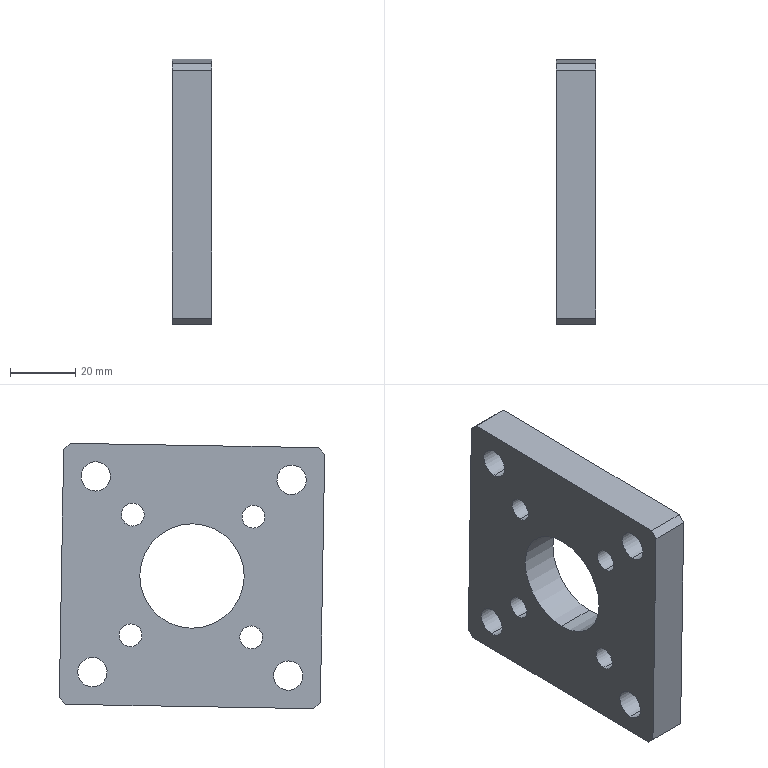Component | SolidWorks | CylinderPlate-1 | 1 solid | 28 faces | box 12 x 81.31 x 81.31 mm | volume 62152 mm3 | cylinder 18 | plane 10 | commonest cylinder face diameters 9 x8 7 x8 32 x2
STEP:
#1=CARTESIAN_POINT('',(37.992,49.965,28.389));
#2=VERTEX_POINT('',#1);
#3=CARTESIAN_POINT('',(37.992,49.971,28.035));
#4=VERTEX_POINT('',#3);
#5=CARTESIAN_POINT('',(37.992,49.968,28.212));
#6=DIRECTION('',(1.,0.,0.));
#7=DIRECTION('',(0.,0.01745,-0.9998));
#8=AXIS2_PLACEMENT_3D('',#5,#6,#7);
#9=CIRCLE('',#8,0.1772);
#10=EDGE_CURVE('',#2,#4,#9,.T.);
#11=ORIENTED_EDGE('',*,*,#10,.T.);
#12=CARTESIAN_POINT('',(37.52,49.971,28.035));
#13=VERTEX_POINT('',#12);
#14=CARTESIAN_POINT('',(37.992,49.971,28.035));
#15=DIRECTION('',(-1.,-0.,-0.));
#16=VECTOR('',#15,39.37);
#17=LINE('',#14,#16);
#18=EDGE_CURVE('',#4,#13,#17,.T.);
#19=ORIENTED_EDGE('',*,*,#18,.T.);
#20=CARTESIAN_POINT('',(37.52,49.965,28.389));
#21=VERTEX_POINT('',#20);
#22=CARTESIAN_POINT('',(37.52,49.968,28.212));
#23=DIRECTION('',(1.,0.,0.));
#24=DIRECTION('',(0.,0.01745,-0.9998));
#25=AXIS2_PLACEMENT_3D('',#22,#23,#24);
#26=CIRCLE('',#25,0.1772);
#27=EDGE_CURVE('',#21,#13,#26,.T.);
#28=ORIENTED_EDGE('',*,*,#27,.F.);
#29=CARTESIAN_POINT('',(37.992,49.965,28.389));
#30=DIRECTION('',(-1.,-0.,-0.));
#31=VECTOR('',#30,39.37);
#32=LINE('',#29,#31);
#33=EDGE_CURVE('',#2,#21,#32,.T.);
#34=ORIENTED_EDGE('',*,*,#33,.F.);
#35=EDGE_LOOP('',(#11,#19,#28,#34));
#36=FACE_OUTER_BOUND('',#35,.T.);
#37=CARTESIAN_POINT('',(37.992,49.968,28.212));
#38=DIRECTION('',(-1.,-0.,-0.));
#39=DIRECTION('',(0.,-0.01745,0.9998));
#40=AXIS2_PLACEMENT_3D('',#37,#38,#39);
#41=CYLINDRICAL_SURFACE('',#40,0.1772);
#42=ADVANCED_FACE('',(#36),#41,.F.);
#43=CARTESIAN_POINT('',(37.992,50.006,26.027));
#44=VERTEX_POINT('',#43);
#45=CARTESIAN_POINT('',(37.992,50.012,25.673));
#46=VERTEX_POINT('',#45);
#47=CARTESIAN_POINT('',(37.992,50.009,25.85));
#48=DIRECTION('',(1.,0.,0.));
#49=DIRECTION('',(0.,0.01745,-0.9998));
#50=AXIS2_PLACEMENT_3D('',#47,#48,#49);
#51=CIRCLE('',#50,0.1772);
#52=EDGE_CURVE('',#44,#46,#51,.T.);
#53=ORIENTED_EDGE('',*,*,#52,.T.);
#54=CARTESIAN_POINT('',(37.52,50.012,25.673));
#55=VERTEX_POINT('',#54);
#56=CARTESIAN_POINT('',(37.992,50.012,25.673));
#57=DIRECTION('',(-1.,-0.,-0.));
#58=VECTOR('',#57,39.37);
#59=LINE('',#56,#58);
#60=EDGE_CURVE('',#46,#55,#59,.T.);
#61=ORIENTED_EDGE('',*,*,#60,.T.);
#62=CARTESIAN_POINT('',(37.52,50.006,26.027));
#63=VERTEX_POINT('',#62);
#64=CARTESIAN_POINT('',(37.52,50.009,25.85));
#65=DIRECTION('',(1.,0.,0.));
#66=DIRECTION('',(0.,0.01745,-0.9998));
#67=AXIS2_PLACEMENT_3D('',#64,#65,#66);
#68=CIRCLE('',#67,0.1772);
#69=EDGE_CURVE('',#63,#55,#68,.T.);
#70=ORIENTED_EDGE('',*,*,#69,.F.);
#71=CARTESIAN_POINT('',(37.992,50.006,26.027));
#72=DIRECTION('',(-1.,-0.,-0.));
#73=VECTOR('',#72,39.37);
#74=LINE('',#71,#73);
#75=EDGE_CURVE('',#44,#63,#74,.T.);
#76=ORIENTED_EDGE('',*,*,#75,.F.);
#77=EDGE_LOOP('',(#53,#61,#70,#76));
#78=FACE_OUTER_BOUND('',#77,.T.);
#79=CARTESIAN_POINT('',(37.992,50.009,25.85));
#80=DIRECTION('',(-1.,-0.,-0.));
#81=DIRECTION('',(0.,-0.01745,0.9998));
#82=AXIS2_PLACEMENT_3D('',#79,#80,#81);
#83=CYLINDRICAL_SURFACE('',#82,0.1772);
#84=ADVANCED_FACE('',(#78),#83,.F.);
#85=CARTESIAN_POINT('',(37.992,52.368,26.069));
#86=VERTEX_POINT('',#85);
#87=CARTESIAN_POINT('',(37.992,52.374,25.714));
#88=VERTEX_POINT('',#87);
#89=CARTESIAN_POINT('',(37.992,52.371,25.891));
#90=DIRECTION('',(1.,0.,0.));
#91=DIRECTION('',(0.,0.01745,-0.9998));
#92=AXIS2_PLACEMENT_3D('',#89,#90,#91);
#93=CIRCLE('',#92,0.1772);
#94=EDGE_CURVE('',#86,#88,#93,.T.);
#95=ORIENTED_EDGE('',*,*,#94,.T.);
#96=CARTESIAN_POINT('',(37.52,52.374,25.714));
#97=VERTEX_POINT('',#96);
#98=CARTESIAN_POINT('',(37.992,52.374,25.714));
#99=DIRECTION('',(-1.,-0.,-0.));
#100=VECTOR('',#99,39.37);
#101=LINE('',#98,#100);
#102=EDGE_CURVE('',#88,#97,#101,.T.);
#103=ORIENTED_EDGE('',*,*,#102,.T.);
#104=CARTESIAN_POINT('',(37.52,52.368,26.069));
#105=VERTEX_POINT('',#104);
#106=CARTESIAN_POINT('',(37.52,52.371,25.891));
#107=DIRECTION('',(1.,0.,0.));
#108=DIRECTION('',(0.,0.01745,-0.9998));
#109=AXIS2_PLACEMENT_3D('',#106,#107,#108);
#110=CIRCLE('',#109,0.1772);
#111=EDGE_CURVE('',#105,#97,#110,.T.);
#112=ORIENTED_EDGE('',*,*,#111,.F.);
#113=CARTESIAN_POINT('',(37.992,52.368,26.069));
#114=DIRECTION('',(-1.,-0.,-0.));
#115=VECTOR('',#114,39.37);
#116=LINE('',#113,#115);
#117=EDGE_CURVE('',#86,#105,#116,.T.);
#118=ORIENTED_EDGE('',*,*,#117,.F.);
#119=EDGE_LOOP('',(#95,#103,#112,#118));
#120=FACE_OUTER_BOUND('',#119,.T.);
#121=CARTESIAN_POINT('',(37.992,52.371,25.891));
#122=DIRECTION('',(-1.,-0.,-0.));
#123=DIRECTION('',(0.,-0.01745,0.9998));
#124=AXIS2_PLACEMENT_3D('',#121,#122,#123);
#125=CYLINDRICAL_SURFACE('',#124,0.1772);
#126=ADVANCED_FACE('',(#120),#125,.F.);
#127=CARTESIAN_POINT('',(37.992,50.426,27.905));
#128=VERTEX_POINT('',#127);
#129=CARTESIAN_POINT('',(37.992,50.431,27.63));
#130=VERTEX_POINT('',#129);
#131=CARTESIAN_POINT('',(37.992,50.429,27.767));
#132=DIRECTION('',(1.,0.,0.));
#133=DIRECTION('',(0.,0.01745,-0.9998));
#134=AXIS2_PLACEMENT_3D('',#131,#132,#133);
#135=CIRCLE('',#134,0.1378);
#136=EDGE_CURVE('',#128,#130,#135,.T.);
#137=ORIENTED_EDGE('',*,*,#136,.T.);
#138=CARTESIAN_POINT('',(37.52,50.431,27.63));
#139=VERTEX_POINT('',#138);
#140=CARTESIAN_POINT('',(37.992,50.431,27.63));
#141=DIRECTION('',(-1.,-0.,-0.));
#142=VECTOR('',#141,39.37);
#143=LINE('',#140,#142);
#144=EDGE_CURVE('',#130,#139,#143,.T.);
#145=ORIENTED_EDGE('',*,*,#144,.T.);
#146=CARTESIAN_POINT('',(37.52,50.426,27.905));
#147=VERTEX_POINT('',#146);
#148=CARTESIAN_POINT('',(37.52,50.429,27.767));
#149=DIRECTION('',(1.,0.,0.));
#150=DIRECTION('',(0.,0.01745,-0.9998));
#151=AXIS2_PLACEMENT_3D('',#148,#149,#150);
#152=CIRCLE('',#151,0.1378);
#153=EDGE_CURVE('',#147,#139,#152,.T.);
#154=ORIENTED_EDGE('',*,*,#153,.F.);
#155=CARTESIAN_POINT('',(37.992,50.426,27.905));
#156=DIRECTION('',(-1.,-0.,-0.));
#157=VECTOR('',#156,39.37);
#158=LINE('',#155,#157);
#159=EDGE_CURVE('',#128,#147,#158,.T.);
#160=ORIENTED_EDGE('',*,*,#159,.F.);
#161=EDGE_LOOP('',(#137,#145,#154,#160));
#162=FACE_OUTER_BOUND('',#161,.T.);
#163=CARTESIAN_POINT('',(37.992,50.429,27.767));
#164=DIRECTION('',(-1.,-0.,-0.));
#165=DIRECTION('',(0.,-0.01745,0.9998));
#166=AXIS2_PLACEMENT_3D('',#163,#164,#165);
#167=CYLINDRICAL_SURFACE('',#166,0.1378);
#168=ADVANCED_FACE('',(#162),#167,.F.);
#169=CARTESIAN_POINT('',(37.992,50.452,26.449));
#170=VERTEX_POINT('',#169);
#171=CARTESIAN_POINT('',(37.992,50.456,26.173));
#172=VERTEX_POINT('',#171);
#173=CARTESIAN_POINT('',(37.992,50.454,26.311));
#174=DIRECTION('',(1.,0.,0.));
#175=DIRECTION('',(0.,0.01745,-0.9998));
#176=AXIS2_PLACEMENT_3D('',#173,#174,#175);
#177=CIRCLE('',#176,0.1378);
#178=EDGE_CURVE('',#170,#172,#177,.T.);
#179=ORIENTED_EDGE('',*,*,#178,.T.);
#180=CARTESIAN_POINT('',(37.52,50.456,26.173));
#181=VERTEX_POINT('',#180);
#182=CARTESIAN_POINT('',(37.992,50.456,26.173));
#183=DIRECTION('',(-1.,-0.,-0.));
#184=VECTOR('',#183,39.37);
#185=LINE('',#182,#184);
#186=EDGE_CURVE('',#172,#181,#185,.T.);
#187=ORIENTED_EDGE('',*,*,#186,.T.);
#188=CARTESIAN_POINT('',(37.52,50.452,26.449));
#189=VERTEX_POINT('',#188);
#190=CARTESIAN_POINT('',(37.52,50.454,26.311));
#191=DIRECTION('',(1.,0.,0.));
#192=DIRECTION('',(0.,0.01745,-0.9998));
#193=AXIS2_PLACEMENT_3D('',#190,#191,#192);
#194=CIRCLE('',#193,0.1378);
#195=EDGE_CURVE('',#189,#181,#194,.T.);
#196=ORIENTED_EDGE('',*,*,#195,.F.);
#197=CARTESIAN_POINT('',(37.992,50.452,26.449));
#198=DIRECTION('',(-1.,-0.,-0.));
#199=VECTOR('',#198,39.37);
#200=LINE('',#197,#199);
#201=EDGE_CURVE('',#170,#189,#200,.T.);
#202=ORIENTED_EDGE('',*,*,#201,.F.);
#203=EDGE_LOOP('',(#179,#187,#196,#202));
#204=FACE_OUTER_BOUND('',#203,.T.);
#205=CARTESIAN_POINT('',(37.992,50.454,26.311));
#206=DIRECTION('',(-1.,-0.,-0.));
#207=DIRECTION('',(0.,-0.01745,0.9998));
#208=AXIS2_PLACEMENT_3D('',#205,#206,#207);
#209=CYLINDRICAL_SURFACE('',#208,0.1378);
#210=ADVANCED_FACE('',(#204),#209,.F.);
#211=CARTESIAN_POINT('',(37.992,51.908,26.474));
#212=VERTEX_POINT('',#211);
#213=CARTESIAN_POINT('',(37.992,51.913,26.199));
#214=VERTEX_POINT('',#213);
#215=CARTESIAN_POINT('',(37.992,51.91,26.336));
#216=DIRECTION('',(1.,0.,0.));
#217=DIRECTION('',(0.,0.01745,-0.9998));
#218=AXIS2_PLACEMENT_3D('',#215,#216,#217);
#219=CIRCLE('',#218,0.1378);
#220=EDGE_CURVE('',#212,#214,#219,.T.);
#221=ORIENTED_EDGE('',*,*,#220,.T.);
#222=CARTESIAN_POINT('',(37.52,51.913,26.199));
#223=VERTEX_POINT('',#222);
#224=CARTESIAN_POINT('',(37.992,51.913,26.199));
#225=DIRECTION('',(-1.,-0.,-0.));
#226=VECTOR('',#225,39.37);
#227=LINE('',#224,#226);
#228=EDGE_CURVE('',#214,#223,#227,.T.);
#229=ORIENTED_EDGE('',*,*,#228,.T.);
#230=CARTESIAN_POINT('',(37.52,51.908,26.474));
#231=VERTEX_POINT('',#230);
#232=CARTESIAN_POINT('',(37.52,51.91,26.336));
#233=DIRECTION('',(1.,0.,0.));
#234=DIRECTION('',(0.,0.01745,-0.9998));
#235=AXIS2_PLACEMENT_3D('',#232,#233,#234);
#236=CIRCLE('',#235,0.1378);
#237=EDGE_CURVE('',#231,#223,#236,.T.);
#238=ORIENTED_EDGE('',*,*,#237,.F.);
#239=CARTESIAN_POINT('',(37.992,51.908,26.474));
#240=DIRECTION('',(-1.,-0.,-0.));
#241=VECTOR('',#240,39.37);
#242=LINE('',#239,#241);
#243=EDGE_CURVE('',#212,#231,#242,.T.);
#244=ORIENTED_EDGE('',*,*,#243,.F.);
#245=EDGE_LOOP('',(#221,#229,#238,#244));
#246=FACE_OUTER_BOUND('',#245,.T.);
#247=CARTESIAN_POINT('',(37.992,51.91,26.336));
#248=DIRECTION('',(-1.,-0.,-0.));
#249=DIRECTION('',(0.,-0.01745,0.9998));
#250=AXIS2_PLACEMENT_3D('',#247,#248,#249);
#251=CYLINDRICAL_SURFACE('',#250,0.1378);
#252=ADVANCED_FACE('',(#246),#251,.F.);
#253=CARTESIAN_POINT('',(37.992,52.327,28.43));
#254=VERTEX_POINT('',#253);
#255=CARTESIAN_POINT('',(37.992,52.333,28.076));
#256=VERTEX_POINT('',#255);
#257=CARTESIAN_POINT('',(37.992,52.33,28.253));
#258=DIRECTION('',(1.,0.,0.));
#259=DIRECTION('',(0.,0.01745,-0.9998));
#260=AXIS2_PLACEMENT_3D('',#257,#258,#259);
#261=CIRCLE('',#260,0.1772);
#262=EDGE_CURVE('',#254,#256,#261,.T.);
#263=ORIENTED_EDGE('',*,*,#262,.T.);
#264=CARTESIAN_POINT('',(37.52,52.333,28.076));
#265=VERTEX_POINT('',#264);
#266=CARTESIAN_POINT('',(37.992,52.333,28.076));
#267=DIRECTION('',(-1.,-0.,-0.));
#268=VECTOR('',#267,39.37);
#269=LINE('',#266,#268);
#270=EDGE_CURVE('',#256,#265,#269,.T.);
#271=ORIENTED_EDGE('',*,*,#270,.T.);
#272=CARTESIAN_POINT('',(37.52,52.327,28.43));
#273=VERTEX_POINT('',#272);
#274=CARTESIAN_POINT('',(37.52,52.33,28.253));
#275=DIRECTION('',(1.,0.,0.));
#276=DIRECTION('',(0.,0.01745,-0.9998));
#277=AXIS2_PLACEMENT_3D('',#274,#275,#276);
#278=CIRCLE('',#277,0.1772);
#279=EDGE_CURVE('',#273,#265,#278,.T.);
#280=ORIENTED_EDGE('',*,*,#279,.F.);
#281=CARTESIAN_POINT('',(37.992,52.327,28.43));
#282=DIRECTION('',(-1.,-0.,-0.));
#283=VECTOR('',#282,39.37);
#284=LINE('',#281,#283);
#285=EDGE_CURVE('',#254,#273,#284,.T.);
#286=ORIENTED_EDGE('',*,*,#285,.F.);
#287=EDGE_LOOP('',(#263,#271,#280,#286));
#288=FACE_OUTER_BOUND('',#287,.T.);
#289=CARTESIAN_POINT('',(37.992,52.33,28.253));
#290=DIRECTION('',(-1.,-0.,-0.));
#291=DIRECTION('',(0.,-0.01745,0.9998));
#292=AXIS2_PLACEMENT_3D('',#289,#290,#291);
#293=CYLINDRICAL_SURFACE('',#292,0.1772);
#294=ADVANCED_FACE('',(#288),#293,.F.);
#295=CARTESIAN_POINT('',(37.992,51.159,27.682));
#296=VERTEX_POINT('',#295);
#297=CARTESIAN_POINT('',(37.992,51.181,26.422));
#298=VERTEX_POINT('',#297);
#299=CARTESIAN_POINT('',(37.992,51.17,27.052));
#300=DIRECTION('',(1.,0.,0.));
#301=DIRECTION('',(0.,0.01745,-0.9998));
#302=AXIS2_PLACEMENT_3D('',#299,#300,#301);
#303=CIRCLE('',#302,0.6299);
#304=EDGE_CURVE('',#296,#298,#303,.T.);
#305=ORIENTED_EDGE('',*,*,#304,.T.);
#306=CARTESIAN_POINT('',(37.52,51.181,26.422));
#307=VERTEX_POINT('',#306);
#308=CARTESIAN_POINT('',(37.992,51.181,26.422));
#309=DIRECTION('',(-1.,-0.,-0.));
#310=VECTOR('',#309,39.37);
#311=LINE('',#308,#310);
#312=EDGE_CURVE('',#298,#307,#311,.T.);
#313=ORIENTED_EDGE('',*,*,#312,.T.);
#314=CARTESIAN_POINT('',(37.52,51.159,27.682));
#315=VERTEX_POINT('',#314);
#316=CARTESIAN_POINT('',(37.52,51.17,27.052));
#317=DIRECTION('',(1.,0.,0.));
#318=DIRECTION('',(0.,0.01745,-0.9998));
#319=AXIS2_PLACEMENT_3D('',#316,#317,#318);
#320=CIRCLE('',#319,0.6299);
#321=EDGE_CURVE('',#315,#307,#320,.T.);
#322=ORIENTED_EDGE('',*,*,#321,.F.);
#323=CARTESIAN_POINT('',(37.992,51.159,27.682));
#324=DIRECTION('',(-1.,-0.,-0.));
#325=VECTOR('',#324,39.37);
#326=LINE('',#323,#325);
#327=EDGE_CURVE('',#296,#315,#326,.T.);
#328=ORIENTED_EDGE('',*,*,#327,.F.);
#329=EDGE_LOOP('',(#305,#313,#322,#328));
#330=FACE_OUTER_BOUND('',#329,.T.);
#331=CARTESIAN_POINT('',(37.992,51.17,27.052));
#332=DIRECTION('',(-1.,-0.,-0.));
#333=DIRECTION('',(0.,-0.01745,0.9998));
#334=AXIS2_PLACEMENT_3D('',#331,#332,#333);
#335=CYLINDRICAL_SURFACE('',#334,0.6299);
#336=ADVANCED_FACE('',(#330),#335,.F.);
#337=CARTESIAN_POINT('',(37.992,51.883,27.931));
#338=VERTEX_POINT('',#337);
#339=CARTESIAN_POINT('',(37.992,51.887,27.655));
#340=VERTEX_POINT('',#339);
#341=CARTESIAN_POINT('',(37.992,51.885,27.793));
#342=DIRECTION('',(1.,0.,0.));
#343=DIRECTION('',(0.,0.01745,-0.9998));
#344=AXIS2_PLACEMENT_3D('',#341,#342,#343);
#345=CIRCLE('',#344,0.1378);
#346=EDGE_CURVE('',#338,#340,#345,.T.);
#347=ORIENTED_EDGE('',*,*,#346,.T.);
#348=CARTESIAN_POINT('',(37.52,51.887,27.655));
#349=VERTEX_POINT('',#348);
#350=CARTESIAN_POINT('',(37.992,51.887,27.655));
#351=DIRECTION('',(-1.,-0.,-0.));
#352=VECTOR('',#351,39.37);
#353=LINE('',#350,#352);
#354=EDGE_CURVE('',#340,#349,#353,.T.);
#355=ORIENTED_EDGE('',*,*,#354,.T.);
#356=CARTESIAN_POINT('',(37.52,51.883,27.931));
#357=VERTEX_POINT('',#356);
#358=CARTESIAN_POINT('',(37.52,51.885,27.793));
#359=DIRECTION('',(1.,0.,0.));
#360=DIRECTION('',(0.,0.01745,-0.9998));
#361=AXIS2_PLACEMENT_3D('',#358,#359,#360);
#362=CIRCLE('',#361,0.1378);
#363=EDGE_CURVE('',#357,#349,#362,.T.);
#364=ORIENTED_EDGE('',*,*,#363,.F.);
#365=CARTESIAN_POINT('',(37.992,51.883,27.931));
#366=DIRECTION('',(-1.,-0.,-0.));
#367=VECTOR('',#366,39.37);
#368=LINE('',#365,#367);
#369=EDGE_CURVE('',#338,#357,#368,.T.);
#370=ORIENTED_EDGE('',*,*,#369,.F.);
#371=EDGE_LOOP('',(#347,#355,#364,#370));
#372=FACE_OUTER_BOUND('',#371,.T.);
#373=CARTESIAN_POINT('',(37.992,51.885,27.793));
#374=DIRECTION('',(-1.,-0.,-0.));
#375=DIRECTION('',(0.,-0.01745,0.9998));
#376=AXIS2_PLACEMENT_3D('',#373,#374,#375);
#377=CYLINDRICAL_SURFACE('',#376,0.1378);
#378=ADVANCED_FACE('',(#372),#377,.F.);
#379=ORIENTED_EDGE('',*,*,#52,.F.);
#380=CARTESIAN_POINT('',(37.992,50.009,25.85));
#381=DIRECTION('',(1.,0.,0.));
#382=DIRECTION('',(0.,0.01745,-0.9998));
#383=AXIS2_PLACEMENT_3D('',#380,#381,#382);
#384=CIRCLE('',#383,0.1772);
#385=EDGE_CURVE('',#46,#44,#384,.T.);
#386=ORIENTED_EDGE('',*,*,#385,.F.);
#387=EDGE_LOOP('',(#379,#386));
#388=FACE_BOUND('',#387,.T.);
#389=ORIENTED_EDGE('',*,*,#136,.F.);
#390=CARTESIAN_POINT('',(37.992,50.429,27.767));
#391=DIRECTION('',(1.,0.,0.));
#392=DIRECTION('',(0.,0.01745,-0.9998));
#393=AXIS2_PLACEMENT_3D('',#390,#391,#392);
#394=CIRCLE('',#393,0.1378);
#395=EDGE_CURVE('',#130,#128,#394,.T.);
#396=ORIENTED_EDGE('',*,*,#395,.F.);
#397=EDGE_LOOP('',(#389,#396));
#398=FACE_BOUND('',#397,.T.);
#399=ORIENTED_EDGE('',*,*,#220,.F.);
#400=CARTESIAN_POINT('',(37.992,51.91,26.336));
#401=DIRECTION('',(1.,0.,0.));
#402=DIRECTION('',(0.,0.01745,-0.9998));
#403=AXIS2_PLACEMENT_3D('',#400,#401,#402);
#404=CIRCLE('',#403,0.1378);
#405=EDGE_CURVE('',#214,#212,#404,.T.);
#406=ORIENTED_EDGE('',*,*,#405,.F.);
#407=EDGE_LOOP('',(#399,#406));
#408=FACE_BOUND('',#407,.T.);
#409=ORIENTED_EDGE('',*,*,#304,.F.);
#410=CARTESIAN_POINT('',(37.992,51.17,27.052));
#411=DIRECTION('',(1.,0.,0.));
#412=DIRECTION('',(0.,0.01745,-0.9998));
#413=AXIS2_PLACEMENT_3D('',#410,#411,#412);
#414=CIRCLE('',#413,0.6299);
#415=EDGE_CURVE('',#298,#296,#414,.T.);
#416=ORIENTED_EDGE('',*,*,#415,.F.);
#417=EDGE_LOOP('',(#409,#416));
#418=FACE_BOUND('',#417,.T.);
#419=CARTESIAN_POINT('',(37.992,52.638,28.652));
#420=VERTEX_POINT('',#419);
#421=CARTESIAN_POINT('',(37.992,49.646,28.6));
#422=VERTEX_POINT('',#421);
#423=CARTESIAN_POINT('',(37.992,52.717,28.654));
#424=DIRECTION('',(0.,-0.9998,-0.01745));
#425=VECTOR('',#424,39.37);
#426=LINE('',#423,#425);
#427=EDGE_CURVE('',#420,#422,#426,.T.);
#428=ORIENTED_EDGE('',*,*,#427,.T.);
#429=CARTESIAN_POINT('',(37.992,49.569,28.52));
#430=VERTEX_POINT('',#429);
#431=CARTESIAN_POINT('',(37.992,49.608,28.56));
#432=DIRECTION('',(0.,-0.6947,-0.7193));
#433=VECTOR('',#432,39.37);
#434=LINE('',#431,#433);
#435=EDGE_CURVE('',#422,#430,#434,.T.);
#436=ORIENTED_EDGE('',*,*,#435,.T.);
#437=CARTESIAN_POINT('',(37.992,49.621,25.528));
#438=VERTEX_POINT('',#437);
#439=CARTESIAN_POINT('',(37.992,49.567,28.599));
#440=DIRECTION('',(-0.,0.01745,-0.9998));
#441=VECTOR('',#440,39.37);
#442=LINE('',#439,#441);
#443=EDGE_CURVE('',#430,#438,#442,.T.);
#444=ORIENTED_EDGE('',*,*,#443,.T.);
#445=CARTESIAN_POINT('',(37.992,49.701,25.451));
#446=VERTEX_POINT('',#445);
#447=CARTESIAN_POINT('',(37.992,49.661,25.49));
#448=DIRECTION('',(-0.,0.7193,-0.6947));
#449=VECTOR('',#448,39.37);
#450=LINE('',#447,#449);
#451=EDGE_CURVE('',#438,#446,#450,.T.);
#452=ORIENTED_EDGE('',*,*,#451,.T.);
#453=CARTESIAN_POINT('',(37.992,52.693,25.503));
#454=VERTEX_POINT('',#453);
#455=CARTESIAN_POINT('',(37.992,52.772,25.505));
#456=DIRECTION('',(-0.,0.9998,0.01745));
#457=VECTOR('',#456,39.37);
#458=LINE('',#455,#457);
#459=EDGE_CURVE('',#446,#454,#458,.T.);
#460=ORIENTED_EDGE('',*,*,#459,.T.);
#461=CARTESIAN_POINT('',(37.992,52.77,25.583));
#462=VERTEX_POINT('',#461);
#463=CARTESIAN_POINT('',(37.992,52.732,25.543));
#464=DIRECTION('',(-0.,0.6947,0.7193));
#465=VECTOR('',#464,39.37);
#466=LINE('',#463,#465);
#467=EDGE_CURVE('',#454,#462,#466,.T.);
#468=ORIENTED_EDGE('',*,*,#467,.T.);
#469=CARTESIAN_POINT('',(37.992,52.718,28.575));
#470=VERTEX_POINT('',#469);
#471=CARTESIAN_POINT('',(37.992,52.717,28.654));
#472=DIRECTION('',(0.,-0.01745,0.9998));
#473=VECTOR('',#472,39.37);
#474=LINE('',#471,#473);
#475=EDGE_CURVE('',#462,#470,#474,.T.);
#476=ORIENTED_EDGE('',*,*,#475,.T.);
#477=CARTESIAN_POINT('',(37.992,52.678,28.614));
#478=DIRECTION('',(0.,-0.7193,0.6947));
#479=VECTOR('',#478,39.37);
#480=LINE('',#477,#479);
#481=EDGE_CURVE('',#470,#420,#480,.T.);
#482=ORIENTED_EDGE('',*,*,#481,.T.);
#483=EDGE_LOOP('',(#428,#436,#444,#452,#460,#468,#476,#482));
#484=FACE_OUTER_BOUND('',#483,.T.);
#485=ORIENTED_EDGE('',*,*,#346,.F.);
#486=CARTESIAN_POINT('',(37.992,51.885,27.793));
#487=DIRECTION('',(1.,0.,0.));
#488=DIRECTION('',(0.,0.01745,-0.9998));
#489=AXIS2_PLACEMENT_3D('',#486,#487,#488);
#490=CIRCLE('',#489,0.1378);
#491=EDGE_CURVE('',#340,#338,#490,.T.);
#492=ORIENTED_EDGE('',*,*,#491,.F.);
#493=EDGE_LOOP('',(#485,#492));
#494=FACE_BOUND('',#493,.T.);
#495=ORIENTED_EDGE('',*,*,#262,.F.);
#496=CARTESIAN_POINT('',(37.992,52.33,28.253));
#497=DIRECTION('',(1.,0.,0.));
#498=DIRECTION('',(0.,0.01745,-0.9998));
#499=AXIS2_PLACEMENT_3D('',#496,#497,#498);
#500=CIRCLE('',#499,0.1772);
#501=EDGE_CURVE('',#256,#254,#500,.T.);
#502=ORIENTED_EDGE('',*,*,#501,.F.);
#503=EDGE_LOOP('',(#495,#502));
#504=FACE_BOUND('',#503,.T.);
#505=ORIENTED_EDGE('',*,*,#178,.F.);
#506=CARTESIAN_POINT('',(37.992,50.454,26.311));
#507=DIRECTION('',(1.,0.,0.));
#508=DIRECTION('',(0.,0.01745,-0.9998));
#509=AXIS2_PLACEMENT_3D('',#506,#507,#508);
#510=CIRCLE('',#509,0.1378);
#511=EDGE_CURVE('',#172,#170,#510,.T.);
#512=ORIENTED_EDGE('',*,*,#511,.F.);
#513=EDGE_LOOP('',(#505,#512));
#514=FACE_BOUND('',#513,.T.);
#515=ORIENTED_EDGE('',*,*,#94,.F.);
#516=CARTESIAN_POINT('',(37.992,52.371,25.891));
#517=DIRECTION('',(1.,0.,0.));
#518=DIRECTION('',(0.,0.01745,-0.9998));
#519=AXIS2_PLACEMENT_3D('',#516,#517,#518);
#520=CIRCLE('',#519,0.1772);
#521=EDGE_CURVE('',#88,#86,#520,.T.);
#522=ORIENTED_EDGE('',*,*,#521,.F.);
#523=EDGE_LOOP('',(#515,#522));
#524=FACE_BOUND('',#523,.T.);
#525=ORIENTED_EDGE('',*,*,#10,.F.);
#526=CARTESIAN_POINT('',(37.992,49.968,28.212));
#527=DIRECTION('',(1.,0.,0.));
#528=DIRECTION('',(0.,0.01745,-0.9998));
#529=AXIS2_PLACEMENT_3D('',#526,#527,#528);
#530=CIRCLE('',#529,0.1772);
#531=EDGE_CURVE('',#4,#2,#530,.T.);
#532=ORIENTED_EDGE('',*,*,#531,.F.);
#533=EDGE_LOOP('',(#525,#532));
#534=FACE_BOUND('',#533,.T.);
#535=CARTESIAN_POINT('',(37.992,51.17,27.052));
#536=DIRECTION('',(1.,0.,0.));
#537=DIRECTION('',(-0.,0.01745,-0.9998));
#538=AXIS2_PLACEMENT_3D('',#535,#536,#537);
#539=PLANE('',#538);
#540=ADVANCED_FACE('',(#388,#398,#408,#418,#484,#494,#504,#514,#524,#534),#539,.T.);
#541=CARTESIAN_POINT('',(37.52,49.569,28.52));
#542=VERTEX_POINT('',#541);
#543=CARTESIAN_POINT('',(37.52,49.621,25.528));
#544=VERTEX_POINT('',#543);
#545=CARTESIAN_POINT('',(37.52,49.567,28.599));
#546=DIRECTION('',(-0.,0.01745,-0.9998));
#547=VECTOR('',#546,39.37);
#548=LINE('',#545,#547);
#549=EDGE_CURVE('',#542,#544,#548,.T.);
#550=ORIENTED_EDGE('',*,*,#549,.F.);
#551=CARTESIAN_POINT('',(37.52,49.646,28.6));
#552=VERTEX_POINT('',#551);
#553=CARTESIAN_POINT('',(37.52,49.569,28.52));
#554=DIRECTION('',(-0.,0.6947,0.7193));
#555=VECTOR('',#554,39.37);
#556=LINE('',#553,#555);
#557=EDGE_CURVE('',#542,#552,#556,.T.);
#558=ORIENTED_EDGE('',*,*,#557,.T.);
#559=CARTESIAN_POINT('',(37.52,52.638,28.652));
#560=VERTEX_POINT('',#559);
#561=CARTESIAN_POINT('',(37.52,52.717,28.654));
#562=DIRECTION('',(0.,-0.9998,-0.01745));
#563=VECTOR('',#562,39.37);
#564=LINE('',#561,#563);
#565=EDGE_CURVE('',#560,#552,#564,.T.);
#566=ORIENTED_EDGE('',*,*,#565,.F.);
#567=CARTESIAN_POINT('',(37.52,52.718,28.575));
#568=VERTEX_POINT('',#567);
#569=CARTESIAN_POINT('',(37.52,52.638,28.652));
#570=DIRECTION('',(-0.,0.7193,-0.6947));
#571=VECTOR('',#570,39.37);
#572=LINE('',#569,#571);
#573=EDGE_CURVE('',#560,#568,#572,.T.);
#574=ORIENTED_EDGE('',*,*,#573,.T.);
#575=CARTESIAN_POINT('',(37.52,52.77,25.583));
#576=VERTEX_POINT('',#575);
#577=CARTESIAN_POINT('',(37.52,52.717,28.654));
#578=DIRECTION('',(0.,-0.01745,0.9998));
#579=VECTOR('',#578,39.37);
#580=LINE('',#577,#579);
#581=EDGE_CURVE('',#576,#568,#580,.T.);
#582=ORIENTED_EDGE('',*,*,#581,.F.);
#583=CARTESIAN_POINT('',(37.52,52.693,25.503));
#584=VERTEX_POINT('',#583);
#585=CARTESIAN_POINT('',(37.52,52.77,25.583));
#586=DIRECTION('',(0.,-0.6947,-0.7193));
#587=VECTOR('',#586,39.37);
#588=LINE('',#585,#587);
#589=EDGE_CURVE('',#576,#584,#588,.T.);
#590=ORIENTED_EDGE('',*,*,#589,.T.);
#591=CARTESIAN_POINT('',(37.52,49.701,25.451));
#592=VERTEX_POINT('',#591);
#593=CARTESIAN_POINT('',(37.52,52.772,25.505));
#594=DIRECTION('',(-0.,0.9998,0.01745));
#595=VECTOR('',#594,39.37);
#596=LINE('',#593,#595);
#597=EDGE_CURVE('',#592,#584,#596,.T.);
#598=ORIENTED_EDGE('',*,*,#597,.F.);
#599=CARTESIAN_POINT('',(37.52,49.701,25.451));
#600=DIRECTION('',(0.,-0.7193,0.6947));
#601=VECTOR('',#600,39.37);
#602=LINE('',#599,#601);
#603=EDGE_CURVE('',#592,#544,#602,.T.);
#604=ORIENTED_EDGE('',*,*,#603,.T.);
#605=EDGE_LOOP('',(#550,#558,#566,#574,#582,#590,#598,#604));
#606=FACE_OUTER_BOUND('',#605,.T.);
#607=ORIENTED_EDGE('',*,*,#363,.T.);
#608=CARTESIAN_POINT('',(37.52,51.885,27.793));
#609=DIRECTION('',(1.,0.,0.));
#610=DIRECTION('',(0.,0.01745,-0.9998));
#611=AXIS2_PLACEMENT_3D('',#608,#609,#610);
#612=CIRCLE('',#611,0.1378);
#613=EDGE_CURVE('',#349,#357,#612,.T.);
#614=ORIENTED_EDGE('',*,*,#613,.T.);
#615=EDGE_LOOP('',(#607,#614));
#616=FACE_BOUND('',#615,.T.);
#617=ORIENTED_EDGE('',*,*,#321,.T.);
#618=CARTESIAN_POINT('',(37.52,51.17,27.052));
#619=DIRECTION('',(1.,0.,0.));
#620=DIRECTION('',(0.,0.01745,-0.9998));
#621=AXIS2_PLACEMENT_3D('',#618,#619,#620);
#622=CIRCLE('',#621,0.6299);
#623=EDGE_CURVE('',#307,#315,#622,.T.);
#624=ORIENTED_EDGE('',*,*,#623,.T.);
#625=EDGE_LOOP('',(#617,#624));
#626=FACE_BOUND('',#625,.T.);
#627=ORIENTED_EDGE('',*,*,#279,.T.);
#628=CARTESIAN_POINT('',(37.52,52.33,28.253));
#629=DIRECTION('',(1.,0.,0.));
#630=DIRECTION('',(0.,0.01745,-0.9998));
#631=AXIS2_PLACEMENT_3D('',#628,#629,#630);
#632=CIRCLE('',#631,0.1772);
#633=EDGE_CURVE('',#265,#273,#632,.T.);
#634=ORIENTED_EDGE('',*,*,#633,.T.);
#635=EDGE_LOOP('',(#627,#634));
#636=FACE_BOUND('',#635,.T.);
#637=ORIENTED_EDGE('',*,*,#237,.T.);
#638=CARTESIAN_POINT('',(37.52,51.91,26.336));
#639=DIRECTION('',(1.,0.,0.));
#640=DIRECTION('',(0.,0.01745,-0.9998));
#641=AXIS2_PLACEMENT_3D('',#638,#639,#640);
#642=CIRCLE('',#641,0.1378);
#643=EDGE_CURVE('',#223,#231,#642,.T.);
#644=ORIENTED_EDGE('',*,*,#643,.T.);
#645=EDGE_LOOP('',(#637,#644));
#646=FACE_BOUND('',#645,.T.);
#647=ORIENTED_EDGE('',*,*,#195,.T.);
#648=CARTESIAN_POINT('',(37.52,50.454,26.311));
#649=DIRECTION('',(1.,0.,0.));
#650=DIRECTION('',(0.,0.01745,-0.9998));
#651=AXIS2_PLACEMENT_3D('',#648,#649,#650);
#652=CIRCLE('',#651,0.1378);
#653=EDGE_CURVE('',#181,#189,#652,.T.);
#654=ORIENTED_EDGE('',*,*,#653,.T.);
#655=EDGE_LOOP('',(#647,#654));
#656=FACE_BOUND('',#655,.T.);
#657=ORIENTED_EDGE('',*,*,#153,.T.);
#658=CARTESIAN_POINT('',(37.52,50.429,27.767));
#659=DIRECTION('',(1.,0.,0.));
#660=DIRECTION('',(0.,0.01745,-0.9998));
#661=AXIS2_PLACEMENT_3D('',#658,#659,#660);
#662=CIRCLE('',#661,0.1378);
#663=EDGE_CURVE('',#139,#147,#662,.T.);
#664=ORIENTED_EDGE('',*,*,#663,.T.);
#665=EDGE_LOOP('',(#657,#664));
#666=FACE_BOUND('',#665,.T.);
#667=ORIENTED_EDGE('',*,*,#111,.T.);
#668=CARTESIAN_POINT('',(37.52,52.371,25.891));
#669=DIRECTION('',(1.,0.,0.));
#670=DIRECTION('',(0.,0.01745,-0.9998));
#671=AXIS2_PLACEMENT_3D('',#668,#669,#670);
#672=CIRCLE('',#671,0.1772);
#673=EDGE_CURVE('',#97,#105,#672,.T.);
#674=ORIENTED_EDGE('',*,*,#673,.T.);
#675=EDGE_LOOP('',(#667,#674));
#676=FACE_BOUND('',#675,.T.);
#677=ORIENTED_EDGE('',*,*,#69,.T.);
#678=CARTESIAN_POINT('',(37.52,50.009,25.85));
#679=DIRECTION('',(1.,0.,0.));
#680=DIRECTION('',(0.,0.01745,-0.9998));
#681=AXIS2_PLACEMENT_3D('',#678,#679,#680);
#682=CIRCLE('',#681,0.1772);
#683=EDGE_CURVE('',#55,#63,#682,.T.);
#684=ORIENTED_EDGE('',*,*,#683,.T.);
#685=EDGE_LOOP('',(#677,#684));
#686=FACE_BOUND('',#685,.T.);
#687=ORIENTED_EDGE('',*,*,#27,.T.);
#688=CARTESIAN_POINT('',(37.52,49.968,28.212));
#689=DIRECTION('',(1.,0.,0.));
#690=DIRECTION('',(0.,0.01745,-0.9998));
#691=AXIS2_PLACEMENT_3D('',#688,#689,#690);
#692=CIRCLE('',#691,0.1772);
#693=EDGE_CURVE('',#13,#21,#692,.T.);
#694=ORIENTED_EDGE('',*,*,#693,.T.);
#695=EDGE_LOOP('',(#687,#694));
#696=FACE_BOUND('',#695,.T.);
#697=CARTESIAN_POINT('',(37.52,51.17,27.052));
#698=DIRECTION('',(1.,0.,0.));
#699=DIRECTION('',(-0.,0.01745,-0.9998));
#700=AXIS2_PLACEMENT_3D('',#697,#698,#699);
#701=PLANE('',#700);
#702=ADVANCED_FACE('',(#606,#616,#626,#636,#646,#656,#666,#676,#686,#696),#701,.F.);
#703=ORIENTED_EDGE('',*,*,#459,.F.);
#704=CARTESIAN_POINT('',(37.992,49.701,25.451));
#705=DIRECTION('',(-1.,-0.,-0.));
#706=VECTOR('',#705,39.37);
#707=LINE('',#704,#706);
#708=EDGE_CURVE('',#446,#592,#707,.T.);
#709=ORIENTED_EDGE('',*,*,#708,.T.);
#710=ORIENTED_EDGE('',*,*,#597,.T.);
#711=CARTESIAN_POINT('',(37.992,52.693,25.503));
#712=DIRECTION('',(1.,0.,0.));
#713=VECTOR('',#712,39.37);
#714=LINE('',#711,#713);
#715=EDGE_CURVE('',#584,#454,#714,.T.);
#716=ORIENTED_EDGE('',*,*,#715,.T.);
#717=EDGE_LOOP('',(#703,#709,#710,#716));
#718=FACE_OUTER_BOUND('',#717,.T.);
#719=CARTESIAN_POINT('',(37.992,52.772,25.505));
#720=DIRECTION('',(0.,-0.01745,0.9998));
#721=DIRECTION('',(0.,-0.9998,-0.01745));
#722=AXIS2_PLACEMENT_3D('',#719,#720,#721);
#723=PLANE('',#722);
#724=ADVANCED_FACE('',(#718),#723,.F.);
#725=ORIENTED_EDGE('',*,*,#581,.T.);
#726=CARTESIAN_POINT('',(37.992,52.718,28.575));
#727=DIRECTION('',(1.,0.,0.));
#728=VECTOR('',#727,39.37);
#729=LINE('',#726,#728);
#730=EDGE_CURVE('',#568,#470,#729,.T.);
#731=ORIENTED_EDGE('',*,*,#730,.T.);
#732=ORIENTED_EDGE('',*,*,#475,.F.);
#733=CARTESIAN_POINT('',(37.992,52.77,25.583));
#734=DIRECTION('',(-1.,-0.,-0.));
#735=VECTOR('',#734,39.37);
#736=LINE('',#733,#735);
#737=EDGE_CURVE('',#462,#576,#736,.T.);
#738=ORIENTED_EDGE('',*,*,#737,.T.);
#739=EDGE_LOOP('',(#725,#731,#732,#738));
#740=FACE_OUTER_BOUND('',#739,.T.);
#741=CARTESIAN_POINT('',(37.992,52.717,28.654));
#742=DIRECTION('',(0.,-0.9998,-0.01745));
#743=DIRECTION('',(-1.,-0.,-0.));
#744=AXIS2_PLACEMENT_3D('',#741,#742,#743);
#745=PLANE('',#744);
#746=ADVANCED_FACE('',(#740),#745,.F.);
#747=ORIENTED_EDGE('',*,*,#565,.T.);
#748=CARTESIAN_POINT('',(37.992,49.646,28.6));
#749=DIRECTION('',(1.,0.,0.));
#750=VECTOR('',#749,39.37);
#751=LINE('',#748,#750);
#752=EDGE_CURVE('',#552,#422,#751,.T.);
#753=ORIENTED_EDGE('',*,*,#752,.T.);
#754=ORIENTED_EDGE('',*,*,#427,.F.);
#755=CARTESIAN_POINT('',(37.992,52.638,28.652));
#756=DIRECTION('',(-1.,-0.,-0.));
#757=VECTOR('',#756,39.37);
#758=LINE('',#755,#757);
#759=EDGE_CURVE('',#420,#560,#758,.T.);
#760=ORIENTED_EDGE('',*,*,#759,.T.);
#761=EDGE_LOOP('',(#747,#753,#754,#760));
#762=FACE_OUTER_BOUND('',#761,.T.);
#763=CARTESIAN_POINT('',(37.992,52.717,28.654));
#764=DIRECTION('',(-0.,0.01745,-0.9998));
#765=DIRECTION('',(-0.,0.9998,0.01745));
#766=AXIS2_PLACEMENT_3D('',#763,#764,#765);
#767=PLANE('',#766);
#768=ADVANCED_FACE('',(#762),#767,.F.);
#769=ORIENTED_EDGE('',*,*,#443,.F.);
#770=CARTESIAN_POINT('',(37.992,49.569,28.52));
#771=DIRECTION('',(-1.,-0.,-0.));
#772=VECTOR('',#771,39.37);
#773=LINE('',#770,#772);
#774=EDGE_CURVE('',#430,#542,#773,.T.);
#775=ORIENTED_EDGE('',*,*,#774,.T.);
#776=ORIENTED_EDGE('',*,*,#549,.T.);
#777=CARTESIAN_POINT('',(37.992,49.621,25.528));
#778=DIRECTION('',(1.,0.,0.));
#779=VECTOR('',#778,39.37);
#780=LINE('',#777,#779);
#781=EDGE_CURVE('',#544,#438,#780,.T.);
#782=ORIENTED_EDGE('',*,*,#781,.T.);
#783=EDGE_LOOP('',(#769,#775,#776,#782));
#784=FACE_OUTER_BOUND('',#783,.T.);
#785=CARTESIAN_POINT('',(37.992,49.567,28.599));
#786=DIRECTION('',(-0.,0.9998,0.01745));
#787=DIRECTION('',(1.,0.,0.));
#788=AXIS2_PLACEMENT_3D('',#785,#786,#787);
#789=PLANE('',#788);
#790=ADVANCED_FACE('',(#784),#789,.F.);
#791=ORIENTED_EDGE('',*,*,#354,.F.);
#792=ORIENTED_EDGE('',*,*,#491,.T.);
#793=ORIENTED_EDGE('',*,*,#369,.T.);
#794=ORIENTED_EDGE('',*,*,#613,.F.);
#795=EDGE_LOOP('',(#791,#792,#793,#794));
#796=FACE_OUTER_BOUND('',#795,.T.);
#797=CARTESIAN_POINT('',(37.992,51.885,27.793));
#798=DIRECTION('',(-1.,-0.,-0.));
#799=DIRECTION('',(0.,-0.01745,0.9998));
#800=AXIS2_PLACEMENT_3D('',#797,#798,#799);
#801=CYLINDRICAL_SURFACE('',#800,0.1378);
#802=ADVANCED_FACE('',(#796),#801,.F.);
#803=ORIENTED_EDGE('',*,*,#312,.F.);
#804=ORIENTED_EDGE('',*,*,#415,.T.);
#805=ORIENTED_EDGE('',*,*,#327,.T.);
#806=ORIENTED_EDGE('',*,*,#623,.F.);
#807=EDGE_LOOP('',(#803,#804,#805,#806));
#808=FACE_OUTER_BOUND('',#807,.T.);
#809=CARTESIAN_POINT('',(37.992,51.17,27.052));
#810=DIRECTION('',(-1.,-0.,-0.));
#811=DIRECTION('',(0.,-0.01745,0.9998));
#812=AXIS2_PLACEMENT_3D('',#809,#810,#811);
#813=CYLINDRICAL_SURFACE('',#812,0.6299);
#814=ADVANCED_FACE('',(#808),#813,.F.);
#815=ORIENTED_EDGE('',*,*,#270,.F.);
#816=ORIENTED_EDGE('',*,*,#501,.T.);
#817=ORIENTED_EDGE('',*,*,#285,.T.);
#818=ORIENTED_EDGE('',*,*,#633,.F.);
#819=EDGE_LOOP('',(#815,#816,#817,#818));
#820=FACE_OUTER_BOUND('',#819,.T.);
#821=CARTESIAN_POINT('',(37.992,52.33,28.253));
#822=DIRECTION('',(-1.,-0.,-0.));
#823=DIRECTION('',(0.,-0.01745,0.9998));
#824=AXIS2_PLACEMENT_3D('',#821,#822,#823);
#825=CYLINDRICAL_SURFACE('',#824,0.1772);
#826=ADVANCED_FACE('',(#820),#825,.F.);
#827=ORIENTED_EDGE('',*,*,#228,.F.);
#828=ORIENTED_EDGE('',*,*,#405,.T.);
#829=ORIENTED_EDGE('',*,*,#243,.T.);
#830=ORIENTED_EDGE('',*,*,#643,.F.);
#831=EDGE_LOOP('',(#827,#828,#829,#830));
#832=FACE_OUTER_BOUND('',#831,.T.);
#833=CARTESIAN_POINT('',(37.992,51.91,26.336));
#834=DIRECTION('',(-1.,-0.,-0.));
#835=DIRECTION('',(0.,-0.01745,0.9998));
#836=AXIS2_PLACEMENT_3D('',#833,#834,#835);
#837=CYLINDRICAL_SURFACE('',#836,0.1378);
#838=ADVANCED_FACE('',(#832),#837,.F.);
#839=ORIENTED_EDGE('',*,*,#186,.F.);
#840=ORIENTED_EDGE('',*,*,#511,.T.);
#841=ORIENTED_EDGE('',*,*,#201,.T.);
#842=ORIENTED_EDGE('',*,*,#653,.F.);
#843=EDGE_LOOP('',(#839,#840,#841,#842));
#844=FACE_OUTER_BOUND('',#843,.T.);
#845=CARTESIAN_POINT('',(37.992,50.454,26.311));
#846=DIRECTION('',(-1.,-0.,-0.));
#847=DIRECTION('',(0.,-0.01745,0.9998));
#848=AXIS2_PLACEMENT_3D('',#845,#846,#847);
#849=CYLINDRICAL_SURFACE('',#848,0.1378);
#850=ADVANCED_FACE('',(#844),#849,.F.);
#851=ORIENTED_EDGE('',*,*,#144,.F.);
#852=ORIENTED_EDGE('',*,*,#395,.T.);
#853=ORIENTED_EDGE('',*,*,#159,.T.);
#854=ORIENTED_EDGE('',*,*,#663,.F.);
#855=EDGE_LOOP('',(#851,#852,#853,#854));
#856=FACE_OUTER_BOUND('',#855,.T.);
#857=CARTESIAN_POINT('',(37.992,50.429,27.767));
#858=DIRECTION('',(-1.,-0.,-0.));
#859=DIRECTION('',(0.,-0.01745,0.9998));
#860=AXIS2_PLACEMENT_3D('',#857,#858,#859);
#861=CYLINDRICAL_SURFACE('',#860,0.1378);
#862=ADVANCED_FACE('',(#856),#861,.F.);
#863=ORIENTED_EDGE('',*,*,#102,.F.);
#864=ORIENTED_EDGE('',*,*,#521,.T.);
#865=ORIENTED_EDGE('',*,*,#117,.T.);
#866=ORIENTED_EDGE('',*,*,#673,.F.);
#867=EDGE_LOOP('',(#863,#864,#865,#866));
#868=FACE_OUTER_BOUND('',#867,.T.);
#869=CARTESIAN_POINT('',(37.992,52.371,25.891));
#870=DIRECTION('',(-1.,-0.,-0.));
#871=DIRECTION('',(0.,-0.01745,0.9998));
#872=AXIS2_PLACEMENT_3D('',#869,#870,#871);
#873=CYLINDRICAL_SURFACE('',#872,0.1772);
#874=ADVANCED_FACE('',(#868),#873,.F.);
#875=ORIENTED_EDGE('',*,*,#60,.F.);
#876=ORIENTED_EDGE('',*,*,#385,.T.);
#877=ORIENTED_EDGE('',*,*,#75,.T.);
#878=ORIENTED_EDGE('',*,*,#683,.F.);
#879=EDGE_LOOP('',(#875,#876,#877,#878));
#880=FACE_OUTER_BOUND('',#879,.T.);
#881=CARTESIAN_POINT('',(37.992,50.009,25.85));
#882=DIRECTION('',(-1.,-0.,-0.));
#883=DIRECTION('',(0.,-0.01745,0.9998));
#884=AXIS2_PLACEMENT_3D('',#881,#882,#883);
#885=CYLINDRICAL_SURFACE('',#884,0.1772);
#886=ADVANCED_FACE('',(#880),#885,.F.);
#887=ORIENTED_EDGE('',*,*,#18,.F.);
#888=ORIENTED_EDGE('',*,*,#531,.T.);
#889=ORIENTED_EDGE('',*,*,#33,.T.);
#890=ORIENTED_EDGE('',*,*,#693,.F.);
#891=EDGE_LOOP('',(#887,#888,#889,#890));
#892=FACE_OUTER_BOUND('',#891,.T.);
#893=CARTESIAN_POINT('',(37.992,49.968,28.212));
#894=DIRECTION('',(-1.,-0.,-0.));
#895=DIRECTION('',(0.,-0.01745,0.9998));
#896=AXIS2_PLACEMENT_3D('',#893,#894,#895);
#897=CYLINDRICAL_SURFACE('',#896,0.1772);
#898=ADVANCED_FACE('',(#892),#897,.F.);
#899=ORIENTED_EDGE('',*,*,#435,.F.);
#900=ORIENTED_EDGE('',*,*,#752,.F.);
#901=ORIENTED_EDGE('',*,*,#557,.F.);
#902=ORIENTED_EDGE('',*,*,#774,.F.);
#903=EDGE_LOOP('',(#899,#900,#901,#902));
#904=FACE_OUTER_BOUND('',#903,.T.);
#905=CARTESIAN_POINT('',(37.992,49.569,28.52));
#906=DIRECTION('',(-0.,0.7193,-0.6947));
#907=DIRECTION('',(-1.,-0.,-0.));
#908=AXIS2_PLACEMENT_3D('',#905,#906,#907);
#909=PLANE('',#908);
#910=ADVANCED_FACE('',(#904),#909,.F.);
#911=ORIENTED_EDGE('',*,*,#451,.F.);
#912=ORIENTED_EDGE('',*,*,#781,.F.);
#913=ORIENTED_EDGE('',*,*,#603,.F.);
#914=ORIENTED_EDGE('',*,*,#708,.F.);
#915=EDGE_LOOP('',(#911,#912,#913,#914));
#916=FACE_OUTER_BOUND('',#915,.T.);
#917=CARTESIAN_POINT('',(37.992,49.701,25.451));
#918=DIRECTION('',(-0.,0.6947,0.7193));
#919=DIRECTION('',(-1.,-0.,-0.));
#920=AXIS2_PLACEMENT_3D('',#917,#918,#919);
#921=PLANE('',#920);
#922=ADVANCED_FACE('',(#916),#921,.F.);
#923=ORIENTED_EDGE('',*,*,#481,.F.);
#924=ORIENTED_EDGE('',*,*,#730,.F.);
#925=ORIENTED_EDGE('',*,*,#573,.F.);
#926=ORIENTED_EDGE('',*,*,#759,.F.);
#927=EDGE_LOOP('',(#923,#924,#925,#926));
#928=FACE_OUTER_BOUND('',#927,.T.);
#929=CARTESIAN_POINT('',(37.992,52.638,28.652));
#930=DIRECTION('',(0.,-0.6947,-0.7193));
#931=DIRECTION('',(-1.,-0.,-0.));
#932=AXIS2_PLACEMENT_3D('',#929,#930,#931);
#933=PLANE('',#932);
#934=ADVANCED_FACE('',(#928),#933,.F.);
#935=ORIENTED_EDGE('',*,*,#467,.F.);
#936=ORIENTED_EDGE('',*,*,#715,.F.);
#937=ORIENTED_EDGE('',*,*,#589,.F.);
#938=ORIENTED_EDGE('',*,*,#737,.F.);
#939=EDGE_LOOP('',(#935,#936,#937,#938));
#940=FACE_OUTER_BOUND('',#939,.T.);
#941=CARTESIAN_POINT('',(37.992,52.77,25.583));
#942=DIRECTION('',(0.,-0.7193,0.6947));
#943=DIRECTION('',(-1.,-0.,-0.));
#944=AXIS2_PLACEMENT_3D('',#941,#942,#943);
#945=PLANE('',#944);
#946=ADVANCED_FACE('',(#940),#945,.F.);
#947=CLOSED_SHELL('',(#42,#84,#126,#168,#210,#252,#294,#336,#378,#540,#702,#724,#746,#768,#790,#802,#814,#826,#838,#850,#862,#874,#886,#898,#910,#922,#934,#946));
#948=MANIFOLD_SOLID_BREP('',#947);
#949=CARTESIAN_POINT('',(0.,0.,0.));
#950=DIRECTION('',(0.,0.,1.));
#951=DIRECTION('',(1.,0.,0.));
#952=AXIS2_PLACEMENT_3D('',#949,#950,#951);
#953=(LENGTH_UNIT()NAMED_UNIT(*)SI_UNIT($,.METRE.));
#954=LENGTH_MEASURE_WITH_UNIT(LENGTH_MEASURE(0.0254),#953);
#955=DIMENSIONAL_EXPONENTS(1.,0.,0.,0.,0.,0.,0.);
#956=(CONVERSION_BASED_UNIT('',#954)LENGTH_UNIT()NAMED_UNIT(#955));
#957=UNCERTAINTY_MEASURE_WITH_UNIT(LENGTH_MEASURE(0.00001),#956,'','');
#958=(NAMED_UNIT(*)PLANE_ANGLE_UNIT()SI_UNIT($,.RADIAN.));
#959=(NAMED_UNIT(*)SI_UNIT($,.STERADIAN.)SOLID_ANGLE_UNIT());
#960=(GEOMETRIC_REPRESENTATION_CONTEXT(3)GLOBAL_UNCERTAINTY_ASSIGNED_CONTEXT((#957))GLOBAL_UNIT_ASSIGNED_CONTEXT((#956,#958,#959))REPRESENTATION_CONTEXT('',''));
#961=ADVANCED_BREP_SHAPE_REPRESENTATION('',(#948,#952),#960);
#962=COLOUR_RGB('',0.7922,0.8196,0.9333);
#963=FILL_AREA_STYLE_COLOUR('',#962);
#964=FILL_AREA_STYLE('',(#963));
#965=SURFACE_STYLE_FILL_AREA(#964);
#966=SURFACE_SIDE_STYLE('',(#965));
#967=SURFACE_STYLE_USAGE(.BOTH.,#966);
#968=PRESENTATION_STYLE_ASSIGNMENT((#967));
#969=STYLED_ITEM('',(#968),#948);
#970=PRESENTATION_LAYER_ASSIGNMENT('','',(#969));
#971=(LENGTH_UNIT()NAMED_UNIT(*)SI_UNIT($,.METRE.));
#972=LENGTH_MEASURE_WITH_UNIT(LENGTH_MEASURE(0.0254),#971);
#973=DIMENSIONAL_EXPONENTS(1.,0.,0.,0.,0.,0.,0.);
#974=(CONVERSION_BASED_UNIT('',#972)LENGTH_UNIT()NAMED_UNIT(#973));
#975=UNCERTAINTY_MEASURE_WITH_UNIT(LENGTH_MEASURE(0.00001),#974,'','');
#976=(NAMED_UNIT(*)PLANE_ANGLE_UNIT()SI_UNIT($,.RADIAN.));
#977=(NAMED_UNIT(*)SI_UNIT($,.STERADIAN.)SOLID_ANGLE_UNIT());
#978=(GEOMETRIC_REPRESENTATION_CONTEXT(3)GLOBAL_UNCERTAINTY_ASSIGNED_CONTEXT((#975))GLOBAL_UNIT_ASSIGNED_CONTEXT((#974,#976,#977))REPRESENTATION_CONTEXT('',''));
#979=MECHANICAL_DESIGN_GEOMETRIC_PRESENTATION_REPRESENTATION('',(#969),#978);